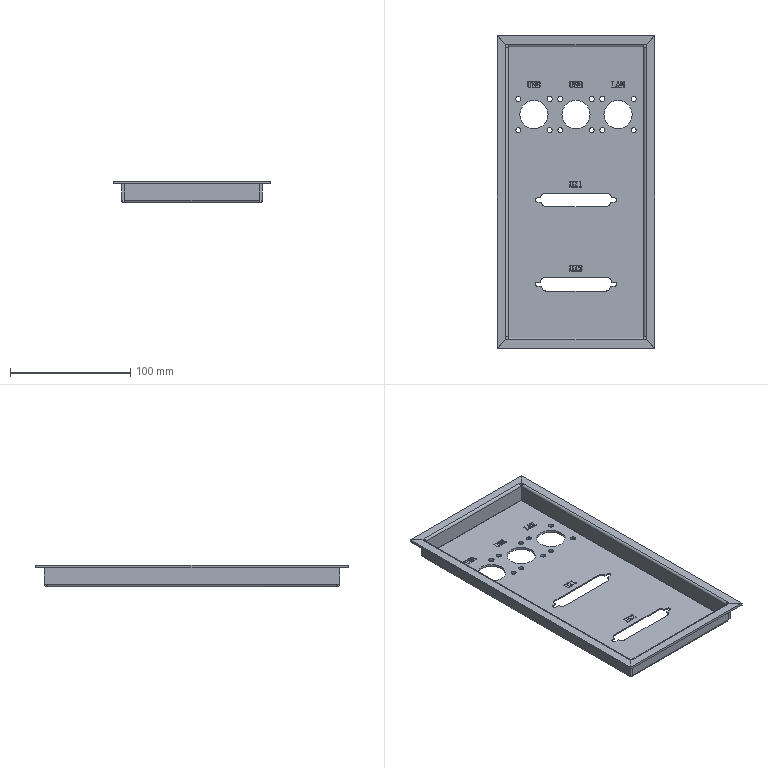CAM job | Mastercam | mm | 6 operations | part box 131 x 260 x 18
1. 2D High Speed (2D Dynamic Mill) | 4 - 4 平铣刀
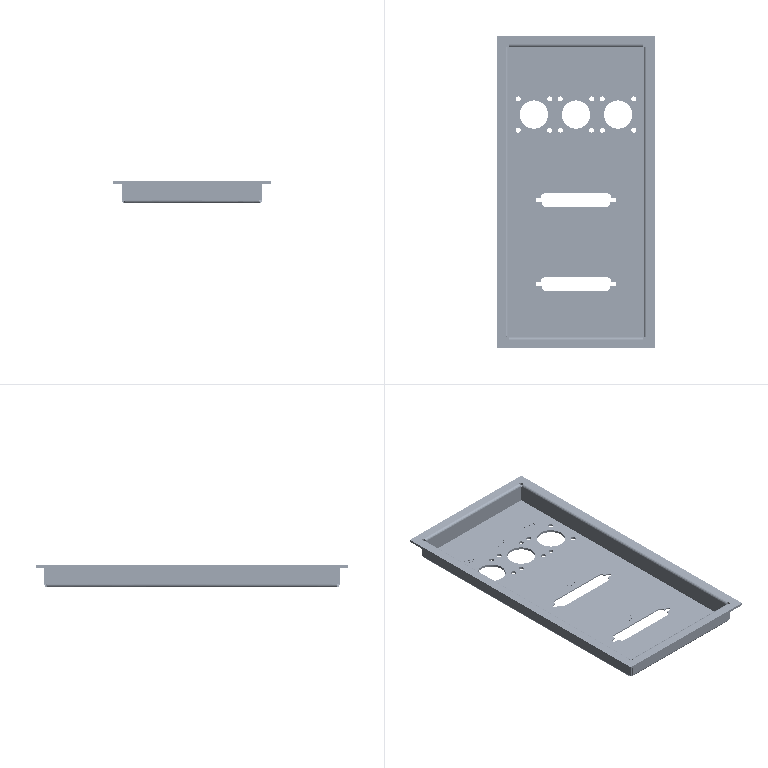2. Contour (2D) | 4 - 4 平铣刀
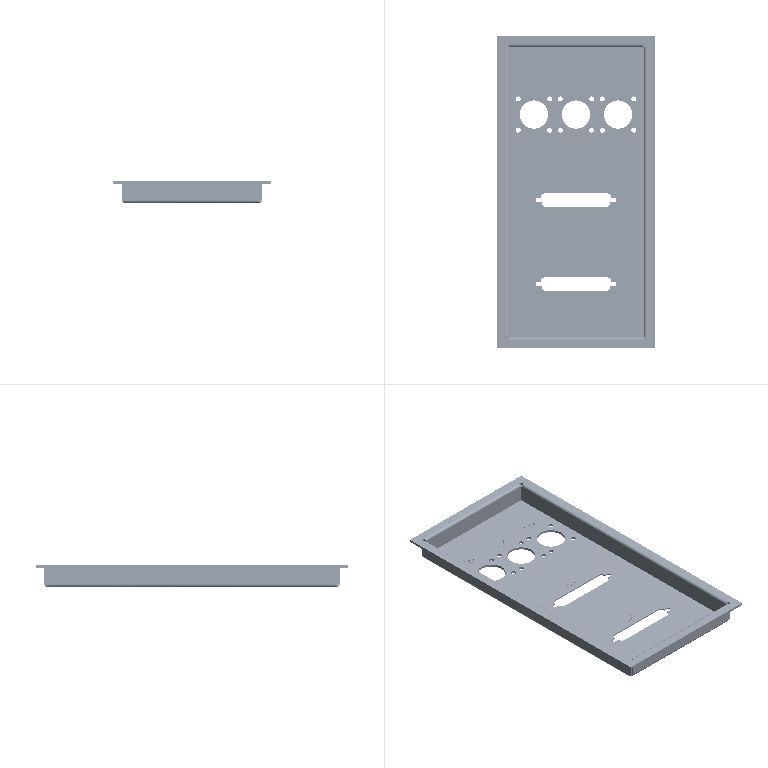3. 3D High Speed (Area roughing) | 3 - 3 平铣刀
4. 2D High Speed (2D Area Mill) | 3 - 3 平铣刀
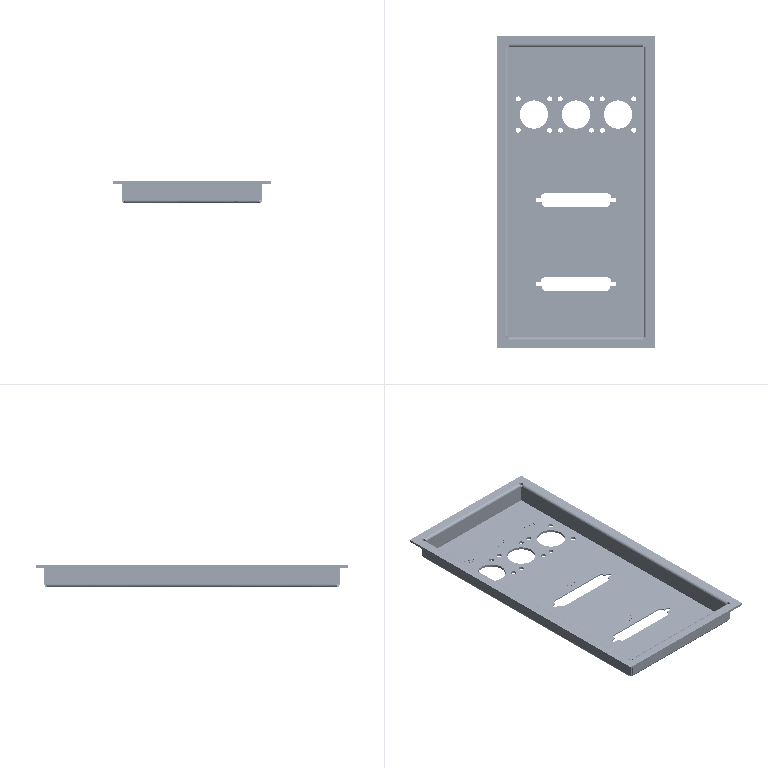5. Contour (2D) | 3 - 3 平铣刀
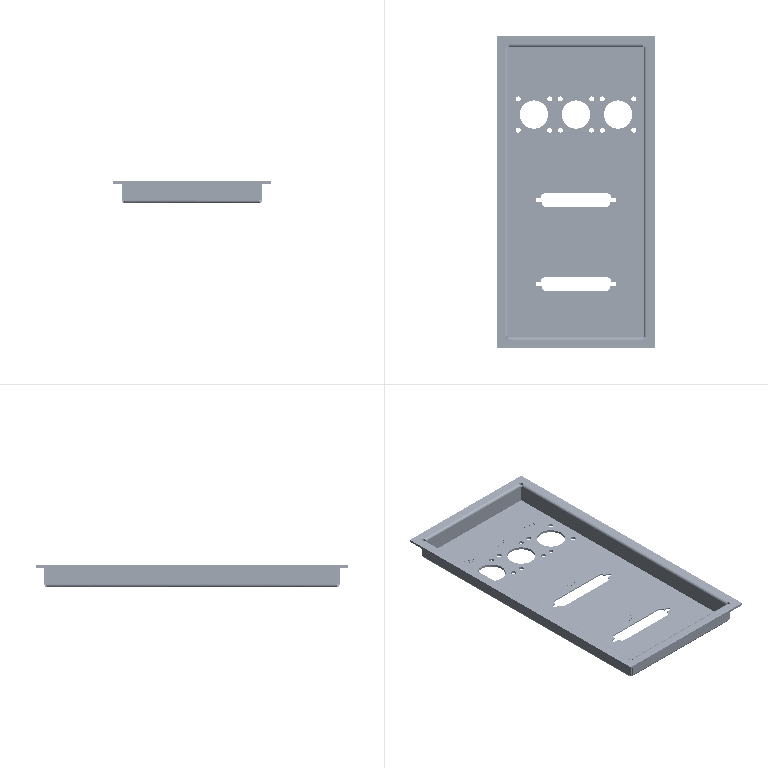6. Drill/Counterbore | 7 - 4 倒角刀